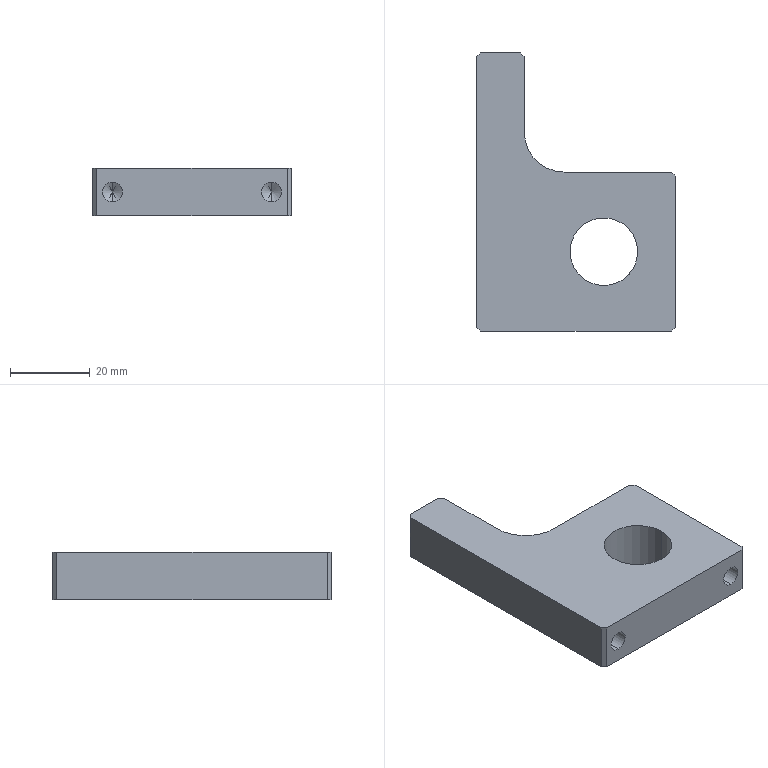Component | SolidWorks | ThirdGenerationFour-sidedLabelingCylinderFixingPlate-1 | 1 solid | 28 faces | box 50 x 70 x 12 mm | volume 24797 mm3 | plane 13 | cylinder 9 | cone 6 | commonest cylinder face diameters 5 x4 4.2 x2 17 x2 20 x1
build123d program:
from build123d import *

# Parameters (mm, degrees)
SKETCH1_W             = 50
SKETCH1_H             = 70
BOSS_EXTRUDE1_DEPTH   = 6
SKETCH4_R             = 8.5
CUT_EXTRUDE1_DEPTH    = 45.654
SKETCH8_W             = 91.952
SKETCH8_H             = 89.251
CUT_EXTRUDE3_DEPTH    = 45.654
M6_TAPPED_HOLE1_D     = 5
M6_TAPPED_HOLE1_DEPTH = 19
M6_TAPPED_HOLE1_TIP   = 1.502
M5_TAPPED_HOLE1_D     = 4.2
M5_TAPPED_HOLE1_DEPTH = 18.4
M5_TAPPED_HOLE1_TIP   = 1.262
CHAMFER1_SIZE         = 1
FILLET1_R             = 10


with BuildPart() as part:
    # Sketch1 → Boss-Extrude1 (new, symmetric)
    with BuildSketch(Plane.XY):
        Rectangle(SKETCH1_W, SKETCH1_H)
    extrude(amount=BOSS_EXTRUDE1_DEPTH, both=True)

    # Sketch4 → Cut-Extrude1 (cut, through all)
    with BuildSketch(Plane(origin=(0, 0, -6), x_dir=(-1, 0, 0), z_dir=(0, 0, -1))):
        with Locations((-7, -15)):
            Circle(SKETCH4_R)
    extrude(amount=-CUT_EXTRUDE1_DEPTH, mode=Mode.SUBTRACT)

    # Sketch8 → Cut-Extrude3 (cut, through all)
    with BuildSketch(Plane(origin=(0, 0, -6), x_dir=(-1, 0, 0), z_dir=(0, 0, -1))):
        with Locations((-32.976, 49.626)):
            Rectangle(SKETCH8_W, SKETCH8_H)
    extrude(amount=-CUT_EXTRUDE3_DEPTH, mode=Mode.SUBTRACT)

    # M6 Tapped Hole1
    with Locations(Plane.XZ.offset(35)):
        with Locations((-20, 0), (20, 0)):
            Hole(M6_TAPPED_HOLE1_D / 2, depth=M6_TAPPED_HOLE1_DEPTH)
            with Locations((0, 0, -(M6_TAPPED_HOLE1_DEPTH + M6_TAPPED_HOLE1_TIP / 2))):  # 118° drill point
                Cone(0, M6_TAPPED_HOLE1_D / 2, M6_TAPPED_HOLE1_TIP, mode=Mode.SUBTRACT)

    # M5 Tapped Hole1
    with Locations(Plane(origin=(0, 35, 0), x_dir=(-1, 0, 0), z_dir=(0, 1, 0))):
        with Locations((19, 0), (89, 0)):
            Hole(M5_TAPPED_HOLE1_D / 2, depth=M5_TAPPED_HOLE1_DEPTH)
            with Locations((0, 0, -(M5_TAPPED_HOLE1_DEPTH + M5_TAPPED_HOLE1_TIP / 2))):  # 118° drill point
                Cone(0, M5_TAPPED_HOLE1_D / 2, M5_TAPPED_HOLE1_TIP, mode=Mode.SUBTRACT)

    # Chamfer1
    chamfer1_edges = [part.edges().sort_by_distance(p)[0] for p in [
        (-13, 35, 0),
        (25, 5, 0),
        (25, -35, 0),
        (-25, -35, 0),
        (-25, 35, 0),
    ]]
    chamfer(chamfer1_edges, length=CHAMFER1_SIZE)

    # Fillet1
    fillet1_edges = [part.edges().sort_by_distance(p)[0] for p in [
        (-13, 5, 0),
    ]]
    fillet(fillet1_edges, radius=FILLET1_R)


solid = part.part

# Placed as in the assembly
solid = solid.moved(Location((52.973, -1.137, -188), (0, 0, 0)))
STEP:
#1=COLOUR_RGB('',0.7922,0.8196,0.9333);
#2=FILL_AREA_STYLE_COLOUR('',#1);
#3=FILL_AREA_STYLE('',(#2));
#4=SURFACE_STYLE_FILL_AREA(#3);
#5=SURFACE_SIDE_STYLE('',(#4));
#6=SURFACE_STYLE_USAGE(.BOTH.,#5);
#7=PRESENTATION_STYLE_ASSIGNMENT((#6));
#8=CARTESIAN_POINT('',(1.338,0.6088,-7.484));
#9=VERTEX_POINT('',#8);
#10=CARTESIAN_POINT('',(1.338,0.6088,-7.319));
#11=VERTEX_POINT('',#10);
#12=CARTESIAN_POINT('',(1.338,0.6088,-7.402));
#13=DIRECTION('',(0.,1.,0.));
#14=DIRECTION('',(0.,0.,1.));
#15=AXIS2_PLACEMENT_3D('',#12,#13,#14);
#16=CIRCLE('',#15,0.08268);
#17=EDGE_CURVE('',#9,#11,#16,.T.);
#18=ORIENTED_EDGE('',*,*,#17,.F.);
#19=CARTESIAN_POINT('',(1.338,1.333,-7.484));
#20=VERTEX_POINT('',#19);
#21=CARTESIAN_POINT('',(1.338,1.333,-7.484));
#22=DIRECTION('',(0.,1.,0.));
#23=VECTOR('',#22,39.37);
#24=LINE('',#21,#23);
#25=EDGE_CURVE('',#9,#20,#24,.T.);
#26=ORIENTED_EDGE('',*,*,#25,.T.);
#27=CARTESIAN_POINT('',(1.338,1.333,-7.319));
#28=VERTEX_POINT('',#27);
#29=CARTESIAN_POINT('',(1.338,1.333,-7.402));
#30=DIRECTION('',(0.,1.,0.));
#31=DIRECTION('',(0.,0.,1.));
#32=AXIS2_PLACEMENT_3D('',#29,#30,#31);
#33=CIRCLE('',#32,0.08268);
#34=EDGE_CURVE('',#20,#28,#33,.T.);
#35=ORIENTED_EDGE('',*,*,#34,.T.);
#36=CARTESIAN_POINT('',(1.338,1.333,-7.319));
#37=DIRECTION('',(0.,1.,0.));
#38=VECTOR('',#37,39.37);
#39=LINE('',#36,#38);
#40=EDGE_CURVE('',#11,#28,#39,.T.);
#41=ORIENTED_EDGE('',*,*,#40,.F.);
#42=EDGE_LOOP('',(#18,#26,#35,#41));
#43=FACE_OUTER_BOUND('',#42,.T.);
#44=CARTESIAN_POINT('',(1.338,1.333,-7.402));
#45=DIRECTION('',(0.,1.,0.));
#46=DIRECTION('',(0.,0.,1.));
#47=AXIS2_PLACEMENT_3D('',#44,#45,#46);
#48=CYLINDRICAL_SURFACE('',#47,0.08268);
#49=ADVANCED_FACE('',(#43),#48,.F.);
#50=CARTESIAN_POINT('',(1.338,0.5591,-7.402));
#51=VERTEX_POINT('',#50);
#52=CARTESIAN_POINT('',(1.338,0.6088,-7.319));
#53=DIRECTION('',(0.,0.515,0.8572));
#54=VECTOR('',#53,39.37);
#55=LINE('',#52,#54);
#56=EDGE_CURVE('',#51,#11,#55,.T.);
#57=ORIENTED_EDGE('',*,*,#56,.F.);
#58=CARTESIAN_POINT('',(1.338,0.6088,-7.484));
#59=DIRECTION('',(0.,0.515,-0.8572));
#60=VECTOR('',#59,39.37);
#61=LINE('',#58,#60);
#62=EDGE_CURVE('',#51,#9,#61,.T.);
#63=ORIENTED_EDGE('',*,*,#62,.T.);
#64=ORIENTED_EDGE('',*,*,#17,.T.);
#65=EDGE_LOOP('',(#57,#63,#64));
#66=FACE_OUTER_BOUND('',#65,.T.);
#67=CARTESIAN_POINT('',(1.338,0.6088,-7.402));
#68=DIRECTION('',(0.,1.,0.));
#69=DIRECTION('',(0.,0.,1.));
#70=AXIS2_PLACEMENT_3D('',#67,#68,#69);
#71=CONICAL_SURFACE('',#70,0.08268,1.03);
#72=ADVANCED_FACE('',(#66),#71,.F.);
#73=CARTESIAN_POINT('',(1.298,-0.6747,-7.303));
#74=VERTEX_POINT('',#73);
#75=CARTESIAN_POINT('',(1.298,-0.6747,-7.5));
#76=VERTEX_POINT('',#75);
#77=CARTESIAN_POINT('',(1.298,-0.6747,-7.402));
#78=DIRECTION('',(0.,-1.,0.));
#79=DIRECTION('',(0.,0.,-1.));
#80=AXIS2_PLACEMENT_3D('',#77,#78,#79);
#81=CIRCLE('',#80,0.09843);
#82=EDGE_CURVE('',#74,#76,#81,.T.);
#83=ORIENTED_EDGE('',*,*,#82,.F.);
#84=CARTESIAN_POINT('',(1.298,-1.423,-7.303));
#85=VERTEX_POINT('',#84);
#86=CARTESIAN_POINT('',(1.298,-1.423,-7.303));
#87=DIRECTION('',(0.,-1.,0.));
#88=VECTOR('',#87,39.37);
#89=LINE('',#86,#88);
#90=EDGE_CURVE('',#74,#85,#89,.T.);
#91=ORIENTED_EDGE('',*,*,#90,.T.);
#92=CARTESIAN_POINT('',(1.298,-1.423,-7.5));
#93=VERTEX_POINT('',#92);
#94=CARTESIAN_POINT('',(1.298,-1.423,-7.402));
#95=DIRECTION('',(0.,-1.,0.));
#96=DIRECTION('',(0.,0.,-1.));
#97=AXIS2_PLACEMENT_3D('',#94,#95,#96);
#98=CIRCLE('',#97,0.09843);
#99=EDGE_CURVE('',#85,#93,#98,.T.);
#100=ORIENTED_EDGE('',*,*,#99,.T.);
#101=CARTESIAN_POINT('',(1.298,-1.423,-7.5));
#102=DIRECTION('',(0.,-1.,0.));
#103=VECTOR('',#102,39.37);
#104=LINE('',#101,#103);
#105=EDGE_CURVE('',#76,#93,#104,.T.);
#106=ORIENTED_EDGE('',*,*,#105,.F.);
#107=EDGE_LOOP('',(#83,#91,#100,#106));
#108=FACE_OUTER_BOUND('',#107,.T.);
#109=CARTESIAN_POINT('',(1.298,-1.423,-7.402));
#110=DIRECTION('',(0.,-1.,0.));
#111=DIRECTION('',(0.,0.,-1.));
#112=AXIS2_PLACEMENT_3D('',#109,#110,#111);
#113=CYLINDRICAL_SURFACE('',#112,0.09843);
#114=ADVANCED_FACE('',(#108),#113,.F.);
#115=CARTESIAN_POINT('',(1.298,-0.6155,-7.402));
#116=VERTEX_POINT('',#115);
#117=CARTESIAN_POINT('',(1.298,-0.6747,-7.5));
#118=DIRECTION('',(0.,-0.515,-0.8572));
#119=VECTOR('',#118,39.37);
#120=LINE('',#117,#119);
#121=EDGE_CURVE('',#116,#76,#120,.T.);
#122=ORIENTED_EDGE('',*,*,#121,.F.);
#123=CARTESIAN_POINT('',(1.298,-0.6747,-7.303));
#124=DIRECTION('',(0.,-0.515,0.8572));
#125=VECTOR('',#124,39.37);
#126=LINE('',#123,#125);
#127=EDGE_CURVE('',#116,#74,#126,.T.);
#128=ORIENTED_EDGE('',*,*,#127,.T.);
#129=ORIENTED_EDGE('',*,*,#82,.T.);
#130=EDGE_LOOP('',(#122,#128,#129));
#131=FACE_OUTER_BOUND('',#130,.T.);
#132=CARTESIAN_POINT('',(1.298,-0.6747,-7.402));
#133=DIRECTION('',(0.,-1.,0.));
#134=DIRECTION('',(0.,0.,-1.));
#135=AXIS2_PLACEMENT_3D('',#132,#133,#134);
#136=CONICAL_SURFACE('',#135,0.09843,1.03);
#137=ADVANCED_FACE('',(#131),#136,.F.);
#138=CARTESIAN_POINT('',(2.873,-0.6747,-7.303));
#139=VERTEX_POINT('',#138);
#140=CARTESIAN_POINT('',(2.873,-0.6747,-7.5));
#141=VERTEX_POINT('',#140);
#142=CARTESIAN_POINT('',(2.873,-0.6747,-7.402));
#143=DIRECTION('',(0.,-1.,0.));
#144=DIRECTION('',(0.,0.,-1.));
#145=AXIS2_PLACEMENT_3D('',#142,#143,#144);
#146=CIRCLE('',#145,0.09843);
#147=EDGE_CURVE('',#139,#141,#146,.T.);
#148=ORIENTED_EDGE('',*,*,#147,.F.);
#149=CARTESIAN_POINT('',(2.873,-1.423,-7.303));
#150=VERTEX_POINT('',#149);
#151=CARTESIAN_POINT('',(2.873,-1.423,-7.303));
#152=DIRECTION('',(0.,-1.,0.));
#153=VECTOR('',#152,39.37);
#154=LINE('',#151,#153);
#155=EDGE_CURVE('',#139,#150,#154,.T.);
#156=ORIENTED_EDGE('',*,*,#155,.T.);
#157=CARTESIAN_POINT('',(2.873,-1.423,-7.5));
#158=VERTEX_POINT('',#157);
#159=CARTESIAN_POINT('',(2.873,-1.423,-7.402));
#160=DIRECTION('',(0.,-1.,0.));
#161=DIRECTION('',(0.,0.,-1.));
#162=AXIS2_PLACEMENT_3D('',#159,#160,#161);
#163=CIRCLE('',#162,0.09843);
#164=EDGE_CURVE('',#150,#158,#163,.T.);
#165=ORIENTED_EDGE('',*,*,#164,.T.);
#166=CARTESIAN_POINT('',(2.873,-1.423,-7.5));
#167=DIRECTION('',(0.,-1.,0.));
#168=VECTOR('',#167,39.37);
#169=LINE('',#166,#168);
#170=EDGE_CURVE('',#141,#158,#169,.T.);
#171=ORIENTED_EDGE('',*,*,#170,.F.);
#172=EDGE_LOOP('',(#148,#156,#165,#171));
#173=FACE_OUTER_BOUND('',#172,.T.);
#174=CARTESIAN_POINT('',(2.873,-1.423,-7.402));
#175=DIRECTION('',(0.,-1.,0.));
#176=DIRECTION('',(0.,0.,-1.));
#177=AXIS2_PLACEMENT_3D('',#174,#175,#176);
#178=CYLINDRICAL_SURFACE('',#177,0.09843);
#179=ADVANCED_FACE('',(#173),#178,.F.);
#180=CARTESIAN_POINT('',(2.873,-0.6155,-7.402));
#181=VERTEX_POINT('',#180);
#182=CARTESIAN_POINT('',(2.873,-0.6747,-7.5));
#183=DIRECTION('',(0.,-0.515,-0.8572));
#184=VECTOR('',#183,39.37);
#185=LINE('',#182,#184);
#186=EDGE_CURVE('',#181,#141,#185,.T.);
#187=ORIENTED_EDGE('',*,*,#186,.F.);
#188=CARTESIAN_POINT('',(2.873,-0.6747,-7.303));
#189=DIRECTION('',(0.,-0.515,0.8572));
#190=VECTOR('',#189,39.37);
#191=LINE('',#188,#190);
#192=EDGE_CURVE('',#181,#139,#191,.T.);
#193=ORIENTED_EDGE('',*,*,#192,.T.);
#194=ORIENTED_EDGE('',*,*,#147,.T.);
#195=EDGE_LOOP('',(#187,#193,#194));
#196=FACE_OUTER_BOUND('',#195,.T.);
#197=CARTESIAN_POINT('',(2.873,-0.6747,-7.402));
#198=DIRECTION('',(0.,-1.,0.));
#199=DIRECTION('',(0.,0.,-1.));
#200=AXIS2_PLACEMENT_3D('',#197,#198,#199);
#201=CONICAL_SURFACE('',#200,0.09843,1.03);
#202=ADVANCED_FACE('',(#196),#201,.F.);
#203=CARTESIAN_POINT('',(2.696,-0.6353,-7.165));
#204=VERTEX_POINT('',#203);
#205=CARTESIAN_POINT('',(2.027,-0.6353,-7.165));
#206=VERTEX_POINT('',#205);
#207=CARTESIAN_POINT('',(2.361,-0.6353,-7.165));
#208=DIRECTION('',(0.,0.,-1.));
#209=DIRECTION('',(-1.,0.,0.));
#210=AXIS2_PLACEMENT_3D('',#207,#208,#209);
#211=CIRCLE('',#210,0.3346);
#212=EDGE_CURVE('',#204,#206,#211,.T.);
#213=ORIENTED_EDGE('',*,*,#212,.F.);
#214=CARTESIAN_POINT('',(2.696,-0.6353,-7.638));
#215=VERTEX_POINT('',#214);
#216=CARTESIAN_POINT('',(2.696,-0.6353,-7.165));
#217=DIRECTION('',(0.,0.,-1.));
#218=VECTOR('',#217,39.37);
#219=LINE('',#216,#218);
#220=EDGE_CURVE('',#204,#215,#219,.T.);
#221=ORIENTED_EDGE('',*,*,#220,.T.);
#222=CARTESIAN_POINT('',(2.027,-0.6353,-7.638));
#223=VERTEX_POINT('',#222);
#224=CARTESIAN_POINT('',(2.361,-0.6353,-7.638));
#225=DIRECTION('',(0.,0.,-1.));
#226=DIRECTION('',(-1.,0.,0.));
#227=AXIS2_PLACEMENT_3D('',#224,#225,#226);
#228=CIRCLE('',#227,0.3346);
#229=EDGE_CURVE('',#215,#223,#228,.T.);
#230=ORIENTED_EDGE('',*,*,#229,.T.);
#231=CARTESIAN_POINT('',(2.027,-0.6353,-7.165));
#232=DIRECTION('',(0.,0.,-1.));
#233=VECTOR('',#232,39.37);
#234=LINE('',#231,#233);
#235=EDGE_CURVE('',#206,#223,#234,.T.);
#236=ORIENTED_EDGE('',*,*,#235,.F.);
#237=EDGE_LOOP('',(#213,#221,#230,#236));
#238=FACE_OUTER_BOUND('',#237,.T.);
#239=CARTESIAN_POINT('',(2.361,-0.6353,-7.165));
#240=DIRECTION('',(0.,0.,-1.));
#241=DIRECTION('',(-1.,0.,0.));
#242=AXIS2_PLACEMENT_3D('',#239,#240,#241);
#243=CYLINDRICAL_SURFACE('',#242,0.3346);
#244=ADVANCED_FACE('',(#238),#243,.F.);
#245=CARTESIAN_POINT('',(3.07,-1.383,-7.165));
#246=VERTEX_POINT('',#245);
#247=CARTESIAN_POINT('',(3.07,0.1127,-7.165));
#248=VERTEX_POINT('',#247);
#249=CARTESIAN_POINT('',(3.07,-1.423,-7.165));
#250=DIRECTION('',(0.,1.,0.));
#251=VECTOR('',#250,39.37);
#252=LINE('',#249,#251);
#253=EDGE_CURVE('',#246,#248,#252,.T.);
#254=ORIENTED_EDGE('',*,*,#253,.F.);
#255=CARTESIAN_POINT('',(3.07,-1.383,-7.638));
#256=VERTEX_POINT('',#255);
#257=CARTESIAN_POINT('',(3.07,-1.383,-7.165));
#258=DIRECTION('',(0.,0.,-1.));
#259=VECTOR('',#258,39.37);
#260=LINE('',#257,#259);
#261=EDGE_CURVE('',#246,#256,#260,.T.);
#262=ORIENTED_EDGE('',*,*,#261,.T.);
#263=CARTESIAN_POINT('',(3.07,0.1127,-7.638));
#264=VERTEX_POINT('',#263);
#265=CARTESIAN_POINT('',(3.07,-1.423,-7.638));
#266=DIRECTION('',(0.,1.,0.));
#267=VECTOR('',#266,39.37);
#268=LINE('',#265,#267);
#269=EDGE_CURVE('',#256,#264,#268,.T.);
#270=ORIENTED_EDGE('',*,*,#269,.T.);
#271=CARTESIAN_POINT('',(3.07,0.1127,-7.165));
#272=DIRECTION('',(0.,0.,1.));
#273=VECTOR('',#272,39.37);
#274=LINE('',#271,#273);
#275=EDGE_CURVE('',#264,#248,#274,.T.);
#276=ORIENTED_EDGE('',*,*,#275,.T.);
#277=EDGE_LOOP('',(#254,#262,#270,#276));
#278=FACE_OUTER_BOUND('',#277,.T.);
#279=CARTESIAN_POINT('',(3.07,-1.423,-7.165));
#280=DIRECTION('',(-1.,0.,0.));
#281=DIRECTION('',(0.,0.,1.));
#282=AXIS2_PLACEMENT_3D('',#279,#280,#281);
#283=PLANE('',#282);
#284=ADVANCED_FACE('',(#278),#283,.F.);
#285=CARTESIAN_POINT('',(1.338,1.333,-7.402));
#286=DIRECTION('',(0.,1.,0.));
#287=DIRECTION('',(0.,0.,1.));
#288=AXIS2_PLACEMENT_3D('',#285,#286,#287);
#289=CIRCLE('',#288,0.08268);
#290=EDGE_CURVE('',#28,#20,#289,.T.);
#291=ORIENTED_EDGE('',*,*,#290,.F.);
#292=ORIENTED_EDGE('',*,*,#34,.F.);
#293=EDGE_LOOP('',(#291,#292));
#294=FACE_BOUND('',#293,.T.);
#295=CARTESIAN_POINT('',(1.534,1.333,-7.638));
#296=VERTEX_POINT('',#295);
#297=CARTESIAN_POINT('',(1.141,1.333,-7.638));
#298=VERTEX_POINT('',#297);
#299=CARTESIAN_POINT('',(1.101,1.333,-7.638));
#300=DIRECTION('',(-1.,0.,0.));
#301=VECTOR('',#300,39.37);
#302=LINE('',#299,#301);
#303=EDGE_CURVE('',#296,#298,#302,.T.);
#304=ORIENTED_EDGE('',*,*,#303,.T.);
#305=CARTESIAN_POINT('',(1.141,1.333,-7.165));
#306=VERTEX_POINT('',#305);
#307=CARTESIAN_POINT('',(1.141,1.333,-7.165));
#308=DIRECTION('',(0.,0.,1.));
#309=VECTOR('',#308,39.37);
#310=LINE('',#307,#309);
#311=EDGE_CURVE('',#298,#306,#310,.T.);
#312=ORIENTED_EDGE('',*,*,#311,.T.);
#313=CARTESIAN_POINT('',(1.534,1.333,-7.165));
#314=VERTEX_POINT('',#313);
#315=CARTESIAN_POINT('',(1.101,1.333,-7.165));
#316=DIRECTION('',(-1.,0.,0.));
#317=VECTOR('',#316,39.37);
#318=LINE('',#315,#317);
#319=EDGE_CURVE('',#314,#306,#318,.T.);
#320=ORIENTED_EDGE('',*,*,#319,.F.);
#321=CARTESIAN_POINT('',(1.534,1.333,-7.165));
#322=DIRECTION('',(0.,0.,-1.));
#323=VECTOR('',#322,39.37);
#324=LINE('',#321,#323);
#325=EDGE_CURVE('',#314,#296,#324,.T.);
#326=ORIENTED_EDGE('',*,*,#325,.T.);
#327=EDGE_LOOP('',(#304,#312,#320,#326));
#328=FACE_OUTER_BOUND('',#327,.T.);
#329=CARTESIAN_POINT('',(1.101,1.333,-7.165));
#330=DIRECTION('',(0.,-1.,0.));
#331=DIRECTION('',(0.,0.,-1.));
#332=AXIS2_PLACEMENT_3D('',#329,#330,#331);
#333=PLANE('',#332);
#334=ADVANCED_FACE('',(#294,#328),#333,.F.);
#335=CARTESIAN_POINT('',(1.101,1.294,-7.165));
#336=VERTEX_POINT('',#335);
#337=CARTESIAN_POINT('',(1.101,-1.383,-7.165));
#338=VERTEX_POINT('',#337);
#339=CARTESIAN_POINT('',(1.101,-1.423,-7.165));
#340=DIRECTION('',(0.,-1.,0.));
#341=VECTOR('',#340,39.37);
#342=LINE('',#339,#341);
#343=EDGE_CURVE('',#336,#338,#342,.T.);
#344=ORIENTED_EDGE('',*,*,#343,.F.);
#345=CARTESIAN_POINT('',(1.101,1.294,-7.638));
#346=VERTEX_POINT('',#345);
#347=CARTESIAN_POINT('',(1.101,1.294,-7.165));
#348=DIRECTION('',(0.,0.,-1.));
#349=VECTOR('',#348,39.37);
#350=LINE('',#347,#349);
#351=EDGE_CURVE('',#336,#346,#350,.T.);
#352=ORIENTED_EDGE('',*,*,#351,.T.);
#353=CARTESIAN_POINT('',(1.101,-1.383,-7.638));
#354=VERTEX_POINT('',#353);
#355=CARTESIAN_POINT('',(1.101,-1.423,-7.638));
#356=DIRECTION('',(0.,-1.,0.));
#357=VECTOR('',#356,39.37);
#358=LINE('',#355,#357);
#359=EDGE_CURVE('',#346,#354,#358,.T.);
#360=ORIENTED_EDGE('',*,*,#359,.T.);
#361=CARTESIAN_POINT('',(1.101,-1.383,-7.165));
#362=DIRECTION('',(0.,0.,1.));
#363=VECTOR('',#362,39.37);
#364=LINE('',#361,#363);
#365=EDGE_CURVE('',#354,#338,#364,.T.);
#366=ORIENTED_EDGE('',*,*,#365,.T.);
#367=EDGE_LOOP('',(#344,#352,#360,#366));
#368=FACE_OUTER_BOUND('',#367,.T.);
#369=CARTESIAN_POINT('',(1.101,-1.423,-7.165));
#370=DIRECTION('',(1.,0.,0.));
#371=DIRECTION('',(0.,0.,-1.));
#372=AXIS2_PLACEMENT_3D('',#369,#370,#371);
#373=PLANE('',#372);
#374=ADVANCED_FACE('',(#368),#373,.F.);
#375=CARTESIAN_POINT('',(1.298,-1.423,-7.402));
#376=DIRECTION('',(0.,-1.,0.));
#377=DIRECTION('',(0.,0.,-1.));
#378=AXIS2_PLACEMENT_3D('',#375,#376,#377);
#379=CIRCLE('',#378,0.09843);
#380=EDGE_CURVE('',#93,#85,#379,.T.);
#381=ORIENTED_EDGE('',*,*,#380,.F.);
#382=ORIENTED_EDGE('',*,*,#99,.F.);
#383=EDGE_LOOP('',(#381,#382));
#384=FACE_BOUND('',#383,.T.);
#385=CARTESIAN_POINT('',(2.873,-1.423,-7.402));
#386=DIRECTION('',(0.,-1.,0.));
#387=DIRECTION('',(0.,0.,-1.));
#388=AXIS2_PLACEMENT_3D('',#385,#386,#387);
#389=CIRCLE('',#388,0.09843);
#390=EDGE_CURVE('',#158,#150,#389,.T.);
#391=ORIENTED_EDGE('',*,*,#390,.F.);
#392=ORIENTED_EDGE('',*,*,#164,.F.);
#393=EDGE_LOOP('',(#391,#392));
#394=FACE_BOUND('',#393,.T.);
#395=CARTESIAN_POINT('',(1.141,-1.423,-7.165));
#396=VERTEX_POINT('',#395);
#397=CARTESIAN_POINT('',(3.03,-1.423,-7.165));
#398=VERTEX_POINT('',#397);
#399=CARTESIAN_POINT('',(1.101,-1.423,-7.165));
#400=DIRECTION('',(1.,0.,0.));
#401=VECTOR('',#400,39.37);
#402=LINE('',#399,#401);
#403=EDGE_CURVE('',#396,#398,#402,.T.);
#404=ORIENTED_EDGE('',*,*,#403,.F.);
#405=CARTESIAN_POINT('',(1.141,-1.423,-7.638));
#406=VERTEX_POINT('',#405);
#407=CARTESIAN_POINT('',(1.141,-1.423,-7.165));
#408=DIRECTION('',(0.,0.,-1.));
#409=VECTOR('',#408,39.37);
#410=LINE('',#407,#409);
#411=EDGE_CURVE('',#396,#406,#410,.T.);
#412=ORIENTED_EDGE('',*,*,#411,.T.);
#413=CARTESIAN_POINT('',(3.03,-1.423,-7.638));
#414=VERTEX_POINT('',#413);
#415=CARTESIAN_POINT('',(1.101,-1.423,-7.638));
#416=DIRECTION('',(1.,0.,0.));
#417=VECTOR('',#416,39.37);
#418=LINE('',#415,#417);
#419=EDGE_CURVE('',#406,#414,#418,.T.);
#420=ORIENTED_EDGE('',*,*,#419,.T.);
#421=CARTESIAN_POINT('',(3.03,-1.423,-7.165));
#422=DIRECTION('',(0.,0.,1.));
#423=VECTOR('',#422,39.37);
#424=LINE('',#421,#423);
#425=EDGE_CURVE('',#414,#398,#424,.T.);
#426=ORIENTED_EDGE('',*,*,#425,.T.);
#427=EDGE_LOOP('',(#404,#412,#420,#426));
#428=FACE_OUTER_BOUND('',#427,.T.);
#429=CARTESIAN_POINT('',(1.101,-1.423,-7.165));
#430=DIRECTION('',(0.,1.,0.));
#431=DIRECTION('',(0.,0.,1.));
#432=AXIS2_PLACEMENT_3D('',#429,#430,#431);
#433=PLANE('',#432);
#434=ADVANCED_FACE('',(#384,#394,#428),#433,.F.);
#435=CARTESIAN_POINT('',(2.361,-0.6353,-7.165));
#436=DIRECTION('',(0.,0.,-1.));
#437=DIRECTION('',(-1.,0.,0.));
#438=AXIS2_PLACEMENT_3D('',#435,#436,#437);
#439=CIRCLE('',#438,0.3346);
#440=EDGE_CURVE('',#206,#204,#439,.T.);
#441=ORIENTED_EDGE('',*,*,#440,.T.);
#442=ORIENTED_EDGE('',*,*,#212,.T.);
#443=EDGE_LOOP('',(#441,#442));
#444=FACE_BOUND('',#443,.T.);
#445=ORIENTED_EDGE('',*,*,#319,.T.);
#446=CARTESIAN_POINT('',(1.101,1.294,-7.165));
#447=DIRECTION('',(-0.7071,-0.7071,0.));
#448=VECTOR('',#447,39.37);
#449=LINE('',#446,#448);
#450=EDGE_CURVE('',#306,#336,#449,.T.);
#451=ORIENTED_EDGE('',*,*,#450,.T.);
#452=ORIENTED_EDGE('',*,*,#343,.T.);
#453=CARTESIAN_POINT('',(1.141,-1.423,-7.165));
#454=DIRECTION('',(0.7071,-0.7071,0.));
#455=VECTOR('',#454,39.37);
#456=LINE('',#453,#455);
#457=EDGE_CURVE('',#338,#396,#456,.T.);
#458=ORIENTED_EDGE('',*,*,#457,.T.);
#459=ORIENTED_EDGE('',*,*,#403,.T.);
#460=CARTESIAN_POINT('',(3.07,-1.383,-7.165));
#461=DIRECTION('',(0.7071,0.7071,0.));
#462=VECTOR('',#461,39.37);
#463=LINE('',#460,#462);
#464=EDGE_CURVE('',#398,#246,#463,.T.);
#465=ORIENTED_EDGE('',*,*,#464,.T.);
#466=ORIENTED_EDGE('',*,*,#253,.T.);
#467=CARTESIAN_POINT('',(3.03,0.1521,-7.165));
#468=VERTEX_POINT('',#467);
#469=CARTESIAN_POINT('',(3.07,0.1127,-7.165));
#470=DIRECTION('',(-0.7071,0.7071,0.));
#471=VECTOR('',#470,39.37);
#472=LINE('',#469,#471);
#473=EDGE_CURVE('',#248,#468,#472,.T.);
#474=ORIENTED_EDGE('',*,*,#473,.T.);
#475=CARTESIAN_POINT('',(1.967,0.1521,-7.165));
#476=VERTEX_POINT('',#475);
#477=CARTESIAN_POINT('',(5.194,0.1521,-7.165));
#478=DIRECTION('',(-1.,0.,0.));
#479=VECTOR('',#478,39.37);
#480=LINE('',#477,#479);
#481=EDGE_CURVE('',#468,#476,#480,.T.);
#482=ORIENTED_EDGE('',*,*,#481,.T.);
#483=CARTESIAN_POINT('',(1.574,0.5458,-7.165));
#484=VERTEX_POINT('',#483);
#485=CARTESIAN_POINT('',(1.967,0.5458,-7.165));
#486=DIRECTION('',(0.,0.,-1.));
#487=DIRECTION('',(-1.,0.,0.));
#488=AXIS2_PLACEMENT_3D('',#485,#486,#487);
#489=CIRCLE('',#488,0.3937);
#490=EDGE_CURVE('',#476,#484,#489,.T.);
#491=ORIENTED_EDGE('',*,*,#490,.T.);
#492=CARTESIAN_POINT('',(1.574,1.294,-7.165));
#493=VERTEX_POINT('',#492);
#494=CARTESIAN_POINT('',(1.574,3.666,-7.165));
#495=DIRECTION('',(0.,1.,0.));
#496=VECTOR('',#495,39.37);
#497=LINE('',#494,#496);
#498=EDGE_CURVE('',#484,#493,#497,.T.);
#499=ORIENTED_EDGE('',*,*,#498,.T.);
#500=CARTESIAN_POINT('',(1.534,1.333,-7.165));
#501=DIRECTION('',(-0.7071,0.7071,0.));
#502=VECTOR('',#501,39.37);
#503=LINE('',#500,#502);
#504=EDGE_CURVE('',#493,#314,#503,.T.);
#505=ORIENTED_EDGE('',*,*,#504,.T.);
#506=EDGE_LOOP('',(#445,#451,#452,#458,#459,#465,#466,#474,#482,#491,#499,#505));
#507=FACE_OUTER_BOUND('',#506,.T.);
#508=CARTESIAN_POINT('',(3.07,1.333,-7.165));
#509=DIRECTION('',(0.,0.,-1.));
#510=DIRECTION('',(-1.,0.,0.));
#511=AXIS2_PLACEMENT_3D('',#508,#509,#510);
#512=PLANE('',#511);
#513=ADVANCED_FACE('',(#444,#507),#512,.F.);
#514=ORIENTED_EDGE('',*,*,#359,.F.);
#515=CARTESIAN_POINT('',(2.105,2.298,-7.638));
#516=DIRECTION('',(0.7071,0.7071,0.));
#517=VECTOR('',#516,39.37);
#518=LINE('',#515,#517);
#519=EDGE_CURVE('',#346,#298,#518,.T.);
#520=ORIENTED_EDGE('',*,*,#519,.T.);
#521=ORIENTED_EDGE('',*,*,#303,.F.);
#522=CARTESIAN_POINT('',(1.574,1.294,-7.638));
#523=VERTEX_POINT('',#522);
#524=CARTESIAN_POINT('',(2.302,0.5655,-7.638));
#525=DIRECTION('',(0.7071,-0.7071,0.));
#526=VECTOR('',#525,39.37);
#527=LINE('',#524,#526);
#528=EDGE_CURVE('',#296,#523,#527,.T.);
#529=ORIENTED_EDGE('',*,*,#528,.T.);
#530=CARTESIAN_POINT('',(1.574,0.5458,-7.638));
#531=VERTEX_POINT('',#530);
#532=CARTESIAN_POINT('',(1.574,3.666,-7.638));
#533=DIRECTION('',(0.,1.,0.));
#534=VECTOR('',#533,39.37);
#535=LINE('',#532,#534);
#536=EDGE_CURVE('',#531,#523,#535,.T.);
#537=ORIENTED_EDGE('',*,*,#536,.F.);
#538=CARTESIAN_POINT('',(1.967,0.1521,-7.638));
#539=VERTEX_POINT('',#538);
#540=CARTESIAN_POINT('',(1.967,0.5458,-7.638));
#541=DIRECTION('',(0.,0.,1.));
#542=DIRECTION('',(-1.,0.,0.));
#543=AXIS2_PLACEMENT_3D('',#540,#541,#542);
#544=CIRCLE('',#543,0.3937);
#545=EDGE_CURVE('',#531,#539,#544,.T.);
#546=ORIENTED_EDGE('',*,*,#545,.T.);
#547=CARTESIAN_POINT('',(3.03,0.1521,-7.638));
#548=VERTEX_POINT('',#547);
#549=CARTESIAN_POINT('',(3.07,0.1521,-7.638));
#550=DIRECTION('',(-1.,0.,0.));
#551=VECTOR('',#550,39.37);
#552=LINE('',#549,#551);
#553=EDGE_CURVE('',#548,#539,#552,.T.);
#554=ORIENTED_EDGE('',*,*,#553,.F.);
#555=CARTESIAN_POINT('',(2.46,0.723,-7.638));
#556=DIRECTION('',(0.7071,-0.7071,0.));
#557=VECTOR('',#556,39.37);
#558=LINE('',#555,#557);
#559=EDGE_CURVE('',#548,#264,#558,.T.);
#560=ORIENTED_EDGE('',*,*,#559,.T.);
#561=ORIENTED_EDGE('',*,*,#269,.F.);
#562=CARTESIAN_POINT('',(4.428,-0.02507,-7.638));
#563=DIRECTION('',(-0.7071,-0.7071,0.));
#564=VECTOR('',#563,39.37);
#565=LINE('',#562,#564);
#566=EDGE_CURVE('',#256,#414,#565,.T.);
#567=ORIENTED_EDGE('',*,*,#566,.T.);
#568=ORIENTED_EDGE('',*,*,#419,.F.);
#569=CARTESIAN_POINT('',(0.7273,-1.009,-7.638));
#570=DIRECTION('',(-0.7071,0.7071,0.));
#571=VECTOR('',#570,39.37);
#572=LINE('',#569,#571);
#573=EDGE_CURVE('',#406,#354,#572,.T.);
#574=ORIENTED_EDGE('',*,*,#573,.T.);
#575=EDGE_LOOP('',(#514,#520,#521,#529,#537,#546,#554,#560,#561,#567,#568,#574));
#576=FACE_OUTER_BOUND('',#575,.T.);
#577=CARTESIAN_POINT('',(2.361,-0.6353,-7.638));
#578=DIRECTION('',(0.,0.,-1.));
#579=DIRECTION('',(-1.,0.,0.));
#580=AXIS2_PLACEMENT_3D('',#577,#578,#579);
#581=CIRCLE('',#580,0.3346);
#582=EDGE_CURVE('',#223,#215,#581,.T.);
#583=ORIENTED_EDGE('',*,*,#582,.F.);
#584=ORIENTED_EDGE('',*,*,#229,.F.);
#585=EDGE_LOOP('',(#583,#584));
#586=FACE_BOUND('',#585,.T.);
#587=CARTESIAN_POINT('',(3.07,1.333,-7.638));
#588=DIRECTION('',(0.,0.,-1.));
#589=DIRECTION('',(-1.,0.,0.));
#590=AXIS2_PLACEMENT_3D('',#587,#588,#589);
#591=PLANE('',#590);
#592=ADVANCED_FACE('',(#576,#586),#591,.T.);
#593=ORIENTED_EDGE('',*,*,#220,.F.);
#594=ORIENTED_EDGE('',*,*,#440,.F.);
#595=ORIENTED_EDGE('',*,*,#235,.T.);
#596=ORIENTED_EDGE('',*,*,#582,.T.);
#597=EDGE_LOOP('',(#593,#594,#595,#596));
#598=FACE_OUTER_BOUND('',#597,.T.);
#599=CARTESIAN_POINT('',(2.361,-0.6353,-7.165));
#600=DIRECTION('',(0.,0.,-1.));
#601=DIRECTION('',(-1.,0.,0.));
#602=AXIS2_PLACEMENT_3D('',#599,#600,#601);
#603=CYLINDRICAL_SURFACE('',#602,0.3346);
#604=ADVANCED_FACE('',(#598),#603,.F.);
#605=ORIENTED_EDGE('',*,*,#498,.F.);
#606=CARTESIAN_POINT('',(1.574,0.5458,-7.638));
#607=DIRECTION('',(0.,0.,-1.));
#608=VECTOR('',#607,39.37);
#609=LINE('',#606,#608);
#610=EDGE_CURVE('',#484,#531,#609,.T.);
#611=ORIENTED_EDGE('',*,*,#610,.T.);
#612=ORIENTED_EDGE('',*,*,#536,.T.);
#613=CARTESIAN_POINT('',(1.574,1.294,-7.165));
#614=DIRECTION('',(0.,0.,1.));
#615=VECTOR('',#614,39.37);
#616=LINE('',#613,#615);
#617=EDGE_CURVE('',#523,#493,#616,.T.);
#618=ORIENTED_EDGE('',*,*,#617,.T.);
#619=EDGE_LOOP('',(#605,#611,#612,#618));
#620=FACE_OUTER_BOUND('',#619,.T.);
#621=CARTESIAN_POINT('',(1.574,3.666,-7.165));
#622=DIRECTION('',(-1.,0.,0.));
#623=DIRECTION('',(-0.,-1.,0.));
#624=AXIS2_PLACEMENT_3D('',#621,#622,#623);
#625=PLANE('',#624);
#626=ADVANCED_FACE('',(#620),#625,.F.);
#627=ORIENTED_EDGE('',*,*,#553,.T.);
#628=CARTESIAN_POINT('',(1.967,0.1521,-7.165));
#629=DIRECTION('',(0.,0.,1.));
#630=VECTOR('',#629,39.37);
#631=LINE('',#628,#630);
#632=EDGE_CURVE('',#539,#476,#631,.T.);
#633=ORIENTED_EDGE('',*,*,#632,.T.);
#634=ORIENTED_EDGE('',*,*,#481,.F.);
#635=CARTESIAN_POINT('',(3.03,0.1521,-7.165));
#636=DIRECTION('',(0.,0.,-1.));
#637=VECTOR('',#636,39.37);
#638=LINE('',#635,#637);
#639=EDGE_CURVE('',#468,#548,#638,.T.);
#640=ORIENTED_EDGE('',*,*,#639,.T.);
#641=EDGE_LOOP('',(#627,#633,#634,#640));
#642=FACE_OUTER_BOUND('',#641,.T.);
#643=CARTESIAN_POINT('',(5.194,0.1521,-7.165));
#644=DIRECTION('',(0.,-1.,0.));
#645=DIRECTION('',(0.,0.,-1.));
#646=AXIS2_PLACEMENT_3D('',#643,#644,#645);
#647=PLANE('',#646);
#648=ADVANCED_FACE('',(#642),#647,.F.);
#649=ORIENTED_EDGE('',*,*,#192,.F.);
#650=ORIENTED_EDGE('',*,*,#186,.T.);
#651=CARTESIAN_POINT('',(2.873,-0.6747,-7.402));
#652=DIRECTION('',(0.,-1.,0.));
#653=DIRECTION('',(0.,0.,-1.));
#654=AXIS2_PLACEMENT_3D('',#651,#652,#653);
#655=CIRCLE('',#654,0.09843);
#656=EDGE_CURVE('',#141,#139,#655,.T.);
#657=ORIENTED_EDGE('',*,*,#656,.T.);
#658=EDGE_LOOP('',(#649,#650,#657));
#659=FACE_OUTER_BOUND('',#658,.T.);
#660=CARTESIAN_POINT('',(2.873,-0.6747,-7.402));
#661=DIRECTION('',(0.,-1.,0.));
#662=DIRECTION('',(0.,0.,-1.));
#663=AXIS2_PLACEMENT_3D('',#660,#661,#662);
#664=CONICAL_SURFACE('',#663,0.09843,1.03);
#665=ADVANCED_FACE('',(#659),#664,.F.);
#666=ORIENTED_EDGE('',*,*,#155,.F.);
#667=ORIENTED_EDGE('',*,*,#656,.F.);
#668=ORIENTED_EDGE('',*,*,#170,.T.);
#669=ORIENTED_EDGE('',*,*,#390,.T.);
#670=EDGE_LOOP('',(#666,#667,#668,#669));
#671=FACE_OUTER_BOUND('',#670,.T.);
#672=CARTESIAN_POINT('',(2.873,-1.423,-7.402));
#673=DIRECTION('',(0.,-1.,0.));
#674=DIRECTION('',(0.,0.,-1.));
#675=AXIS2_PLACEMENT_3D('',#672,#673,#674);
#676=CYLINDRICAL_SURFACE('',#675,0.09843);
#677=ADVANCED_FACE('',(#671),#676,.F.);
#678=ORIENTED_EDGE('',*,*,#127,.F.);
#679=ORIENTED_EDGE('',*,*,#121,.T.);
#680=CARTESIAN_POINT('',(1.298,-0.6747,-7.402));
#681=DIRECTION('',(0.,-1.,0.));
#682=DIRECTION('',(0.,0.,-1.));
#683=AXIS2_PLACEMENT_3D('',#680,#681,#682);
#684=CIRCLE('',#683,0.09843);
#685=EDGE_CURVE('',#76,#74,#684,.T.);
#686=ORIENTED_EDGE('',*,*,#685,.T.);
#687=EDGE_LOOP('',(#678,#679,#686));
#688=FACE_OUTER_BOUND('',#687,.T.);
#689=CARTESIAN_POINT('',(1.298,-0.6747,-7.402));
#690=DIRECTION('',(0.,-1.,0.));
#691=DIRECTION('',(0.,0.,-1.));
#692=AXIS2_PLACEMENT_3D('',#689,#690,#691);
#693=CONICAL_SURFACE('',#692,0.09843,1.03);
#694=ADVANCED_FACE('',(#688),#693,.F.);
#695=ORIENTED_EDGE('',*,*,#90,.F.);
#696=ORIENTED_EDGE('',*,*,#685,.F.);
#697=ORIENTED_EDGE('',*,*,#105,.T.);
#698=ORIENTED_EDGE('',*,*,#380,.T.);
#699=EDGE_LOOP('',(#695,#696,#697,#698));
#700=FACE_OUTER_BOUND('',#699,.T.);
#701=CARTESIAN_POINT('',(1.298,-1.423,-7.402));
#702=DIRECTION('',(0.,-1.,0.));
#703=DIRECTION('',(0.,0.,-1.));
#704=AXIS2_PLACEMENT_3D('',#701,#702,#703);
#705=CYLINDRICAL_SURFACE('',#704,0.09843);
#706=ADVANCED_FACE('',(#700),#705,.F.);
#707=ORIENTED_EDGE('',*,*,#62,.F.);
#708=ORIENTED_EDGE('',*,*,#56,.T.);
#709=CARTESIAN_POINT('',(1.338,0.6088,-7.402));
#710=DIRECTION('',(0.,1.,0.));
#711=DIRECTION('',(0.,0.,1.));
#712=AXIS2_PLACEMENT_3D('',#709,#710,#711);
#713=CIRCLE('',#712,0.08268);
#714=EDGE_CURVE('',#11,#9,#713,.T.);
#715=ORIENTED_EDGE('',*,*,#714,.T.);
#716=EDGE_LOOP('',(#707,#708,#715));
#717=FACE_OUTER_BOUND('',#716,.T.);
#718=CARTESIAN_POINT('',(1.338,0.6088,-7.402));
#719=DIRECTION('',(0.,1.,0.));
#720=DIRECTION('',(0.,0.,1.));
#721=AXIS2_PLACEMENT_3D('',#718,#719,#720);
#722=CONICAL_SURFACE('',#721,0.08268,1.03);
#723=ADVANCED_FACE('',(#717),#722,.F.);
#724=ORIENTED_EDGE('',*,*,#25,.F.);
#725=ORIENTED_EDGE('',*,*,#714,.F.);
#726=ORIENTED_EDGE('',*,*,#40,.T.);
#727=ORIENTED_EDGE('',*,*,#290,.T.);
#728=EDGE_LOOP('',(#724,#725,#726,#727));
#729=FACE_OUTER_BOUND('',#728,.T.);
#730=CARTESIAN_POINT('',(1.338,1.333,-7.402));
#731=DIRECTION('',(0.,1.,0.));
#732=DIRECTION('',(0.,0.,1.));
#733=AXIS2_PLACEMENT_3D('',#730,#731,#732);
#734=CYLINDRICAL_SURFACE('',#733,0.08268);
#735=ADVANCED_FACE('',(#729),#734,.F.);
#736=ORIENTED_EDGE('',*,*,#450,.F.);
#737=ORIENTED_EDGE('',*,*,#311,.F.);
#738=ORIENTED_EDGE('',*,*,#519,.F.);
#739=ORIENTED_EDGE('',*,*,#351,.F.);
#740=EDGE_LOOP('',(#736,#737,#738,#739));
#741=FACE_OUTER_BOUND('',#740,.T.);
#742=CARTESIAN_POINT('',(1.101,1.294,-7.165));
#743=DIRECTION('',(0.7071,-0.7071,0.));
#744=DIRECTION('',(0.7071,0.7071,0.));
#745=AXIS2_PLACEMENT_3D('',#742,#743,#744);
#746=PLANE('',#745);
#747=ADVANCED_FACE('',(#741),#746,.F.);
#748=ORIENTED_EDGE('',*,*,#504,.F.);
#749=ORIENTED_EDGE('',*,*,#617,.F.);
#750=ORIENTED_EDGE('',*,*,#528,.F.);
#751=ORIENTED_EDGE('',*,*,#325,.F.);
#752=EDGE_LOOP('',(#748,#749,#750,#751));
#753=FACE_OUTER_BOUND('',#752,.T.);
#754=CARTESIAN_POINT('',(1.534,1.333,-7.165));
#755=DIRECTION('',(-0.7071,-0.7071,0.));
#756=DIRECTION('',(0.7071,-0.7071,0.));
#757=AXIS2_PLACEMENT_3D('',#754,#755,#756);
#758=PLANE('',#757);
#759=ADVANCED_FACE('',(#753),#758,.F.);
#760=ORIENTED_EDGE('',*,*,#457,.F.);
#761=ORIENTED_EDGE('',*,*,#365,.F.);
#762=ORIENTED_EDGE('',*,*,#573,.F.);
#763=ORIENTED_EDGE('',*,*,#411,.F.);
#764=EDGE_LOOP('',(#760,#761,#762,#763));
#765=FACE_OUTER_BOUND('',#764,.T.);
#766=CARTESIAN_POINT('',(1.141,-1.423,-7.165));
#767=DIRECTION('',(0.7071,0.7071,0.));
#768=DIRECTION('',(-0.7071,0.7071,0.));
#769=AXIS2_PLACEMENT_3D('',#766,#767,#768);
#770=PLANE('',#769);
#771=ADVANCED_FACE('',(#765),#770,.F.);
#772=ORIENTED_EDGE('',*,*,#464,.F.);
#773=ORIENTED_EDGE('',*,*,#425,.F.);
#774=ORIENTED_EDGE('',*,*,#566,.F.);
#775=ORIENTED_EDGE('',*,*,#261,.F.);
#776=EDGE_LOOP('',(#772,#773,#774,#775));
#777=FACE_OUTER_BOUND('',#776,.T.);
#778=CARTESIAN_POINT('',(3.07,-1.383,-7.165));
#779=DIRECTION('',(-0.7071,0.7071,0.));
#780=DIRECTION('',(-0.7071,-0.7071,0.));
#781=AXIS2_PLACEMENT_3D('',#778,#779,#780);
#782=PLANE('',#781);
#783=ADVANCED_FACE('',(#777),#782,.F.);
#784=ORIENTED_EDGE('',*,*,#559,.F.);
#785=ORIENTED_EDGE('',*,*,#639,.F.);
#786=ORIENTED_EDGE('',*,*,#473,.F.);
#787=ORIENTED_EDGE('',*,*,#275,.F.);
#788=EDGE_LOOP('',(#784,#785,#786,#787));
#789=FACE_OUTER_BOUND('',#788,.T.);
#790=CARTESIAN_POINT('',(3.07,0.1127,-7.165));
#791=DIRECTION('',(-0.7071,-0.7071,0.));
#792=DIRECTION('',(0.7071,-0.7071,0.));
#793=AXIS2_PLACEMENT_3D('',#790,#791,#792);
#794=PLANE('',#793);
#795=ADVANCED_FACE('',(#789),#794,.F.);
#796=ORIENTED_EDGE('',*,*,#490,.F.);
#797=ORIENTED_EDGE('',*,*,#632,.F.);
#798=ORIENTED_EDGE('',*,*,#545,.F.);
#799=ORIENTED_EDGE('',*,*,#610,.F.);
#800=EDGE_LOOP('',(#796,#797,#798,#799));
#801=FACE_OUTER_BOUND('',#800,.T.);
#802=CARTESIAN_POINT('',(1.967,0.5458,-7.165));
#803=DIRECTION('',(0.,0.,1.));
#804=DIRECTION('',(1.,0.,0.));
#805=AXIS2_PLACEMENT_3D('',#802,#803,#804);
#806=CYLINDRICAL_SURFACE('',#805,0.3937);
#807=ADVANCED_FACE('',(#801),#806,.F.);
#808=CLOSED_SHELL('',(#49,#72,#114,#137,#179,#202,#244,#284,#334,#374,#434,#513,#592,#604,#626,#648,#665,#677,#694,#706,#723,#735,#747,#759,#771,#783,#795,#807));
#809=MANIFOLD_SOLID_BREP('',#808);
#810=STYLED_ITEM('',(#7),#809);
#811=(LENGTH_UNIT()NAMED_UNIT(*)SI_UNIT($,.METRE.));
#812=LENGTH_MEASURE_WITH_UNIT(LENGTH_MEASURE(0.0254),#811);
#813=DIMENSIONAL_EXPONENTS(1.,0.,0.,0.,0.,0.,0.);
#814=(CONVERSION_BASED_UNIT('',#812)LENGTH_UNIT()NAMED_UNIT(#813));
#815=UNCERTAINTY_MEASURE_WITH_UNIT(LENGTH_MEASURE(0.00001),#814,'','');
#816=(NAMED_UNIT(*)PLANE_ANGLE_UNIT()SI_UNIT($,.RADIAN.));
#817=(NAMED_UNIT(*)SI_UNIT($,.STERADIAN.)SOLID_ANGLE_UNIT());
#818=(GEOMETRIC_REPRESENTATION_CONTEXT(3)GLOBAL_UNCERTAINTY_ASSIGNED_CONTEXT((#815))GLOBAL_UNIT_ASSIGNED_CONTEXT((#814,#816,#817))REPRESENTATION_CONTEXT('',''));
#819=MECHANICAL_DESIGN_GEOMETRIC_PRESENTATION_REPRESENTATION('',(#810),#818);
#820=PRESENTATION_LAYER_ASSIGNMENT('','',(#810));
#821=CARTESIAN_POINT('',(0.,0.,0.));
#822=DIRECTION('',(0.,0.,1.));
#823=DIRECTION('',(1.,0.,0.));
#824=AXIS2_PLACEMENT_3D('',#821,#822,#823);
#825=(LENGTH_UNIT()NAMED_UNIT(*)SI_UNIT($,.METRE.));
#826=LENGTH_MEASURE_WITH_UNIT(LENGTH_MEASURE(0.0254),#825);
#827=DIMENSIONAL_EXPONENTS(1.,0.,0.,0.,0.,0.,0.);
#828=(CONVERSION_BASED_UNIT('',#826)LENGTH_UNIT()NAMED_UNIT(#827));
#829=UNCERTAINTY_MEASURE_WITH_UNIT(LENGTH_MEASURE(0.00001),#828,'','');
#830=(NAMED_UNIT(*)PLANE_ANGLE_UNIT()SI_UNIT($,.RADIAN.));
#831=(NAMED_UNIT(*)SI_UNIT($,.STERADIAN.)SOLID_ANGLE_UNIT());
#832=(GEOMETRIC_REPRESENTATION_CONTEXT(3)GLOBAL_UNCERTAINTY_ASSIGNED_CONTEXT((#829))GLOBAL_UNIT_ASSIGNED_CONTEXT((#828,#830,#831))REPRESENTATION_CONTEXT('',''));
#833=ADVANCED_BREP_SHAPE_REPRESENTATION('',(#809,#824),#832);